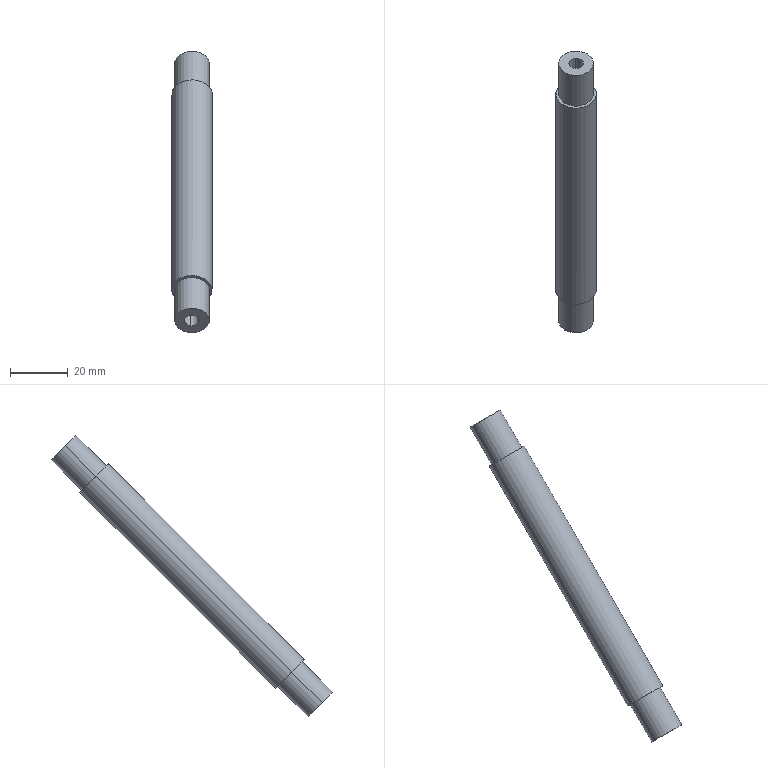Component | SolidWorks | SmallAxisAssembly-1_SmallAxisAssembly1-2_VegetablePressSmallAxis-1 | 1 solid | 18 faces | box 14.05 x 97.58 x 97.58 mm | volume 17562 mm3 | cylinder 10 | cone 4 | plane 4 | commonest cylinder face diameters 5 x4 12 x4 14 x2
build123d program:
from build123d import *

# Parameters (mm, degrees)
M6_TAPPED_HOLE1_D               = 5
M6_TAPPED_HOLE1_DEPTH           = 15
M6_TAPPED_HOLE1_TIP             = 1.502
M6_TAPPED_HOLE1_ON_FACE_2_D     = 5
M6_TAPPED_HOLE1_ON_FACE_2_DEPTH = 15
M6_TAPPED_HOLE1_ON_FACE_2_TIP   = 1.502


with BuildPart() as part:
    # Sketch1 → Revolve1 (revolve)
    with BuildSketch(Plane.XY):
        Polygon((-63, 0), (-63, 6), (-48, 6), (-48, 7), (48, 7), (48, 6), (63, 6), (63, 0), align=None)
    revolve(axis=Axis((63, 0, 0), (-1, 0, 0)))

    # M6 Tapped Hole1
    with Locations(Plane(origin=(63, 0, 0), x_dir=(0, 0, 1), z_dir=(1, 0, 0))):
        with Locations((0, 0)):
            Hole(M6_TAPPED_HOLE1_D / 2, depth=M6_TAPPED_HOLE1_DEPTH)
            with Locations((0, 0, -(M6_TAPPED_HOLE1_DEPTH + M6_TAPPED_HOLE1_TIP / 2))):  # 118° drill point
                Cone(0, M6_TAPPED_HOLE1_D / 2, M6_TAPPED_HOLE1_TIP, mode=Mode.SUBTRACT)

    # M6 Tapped Hole1 on face 2
    with Locations(Plane(origin=(-63, 0, 0), x_dir=(0, 0, -1), z_dir=(-1, 0, 0))):
        with Locations((0, 0)):
            Hole(M6_TAPPED_HOLE1_ON_FACE_2_D / 2, depth=M6_TAPPED_HOLE1_ON_FACE_2_DEPTH)
            with Locations((0, 0, -(M6_TAPPED_HOLE1_ON_FACE_2_DEPTH + M6_TAPPED_HOLE1_ON_FACE_2_TIP / 2))):  # 118° drill point
                Cone(0, M6_TAPPED_HOLE1_ON_FACE_2_D / 2, M6_TAPPED_HOLE1_ON_FACE_2_TIP, mode=Mode.SUBTRACT)


solid = part.part

# Placed as in the assembly
solid = solid.moved(Location((-41.751, 822.318, 226.866), (-135.031, 46.235, -89.957)))
STEP:
#1=COLOUR_RGB('',0.7922,0.8196,0.9333);
#2=FILL_AREA_STYLE_COLOUR('',#1);
#3=FILL_AREA_STYLE('',(#2));
#4=SURFACE_STYLE_FILL_AREA(#3);
#5=SURFACE_SIDE_STYLE('',(#4));
#6=SURFACE_STYLE_USAGE(.BOTH.,#5);
#7=PRESENTATION_STYLE_ASSIGNMENT((#6));
#8=CARTESIAN_POINT('',(-1.657,33.78,10.199));
#9=VERTEX_POINT('',#8);
#10=CARTESIAN_POINT('',(-1.628,33.642,10.337));
#11=VERTEX_POINT('',#10);
#12=CARTESIAN_POINT('',(-1.643,33.711,10.268));
#13=DIRECTION('',(0.0005225,0.7071,0.7071));
#14=DIRECTION('',(0.1474,-0.6994,0.6993));
#15=AXIS2_PLACEMENT_3D('',#12,#13,#14);
#16=CIRCLE('',#15,0.09843);
#17=EDGE_CURVE('',#9,#11,#16,.T.);
#18=ORIENTED_EDGE('',*,*,#17,.F.);
#19=CARTESIAN_POINT('',(-1.657,34.197,10.617));
#20=VERTEX_POINT('',#19);
#21=CARTESIAN_POINT('',(-1.657,34.197,10.617));
#22=DIRECTION('',(0.0005225,0.7071,0.7071));
#23=VECTOR('',#22,39.37);
#24=LINE('',#21,#23);
#25=EDGE_CURVE('',#9,#20,#24,.T.);
#26=ORIENTED_EDGE('',*,*,#25,.T.);
#27=CARTESIAN_POINT('',(-1.628,34.06,10.754));
#28=VERTEX_POINT('',#27);
#29=CARTESIAN_POINT('',(-1.642,34.129,10.686));
#30=DIRECTION('',(0.0005225,0.7071,0.7071));
#31=DIRECTION('',(0.1474,-0.6994,0.6993));
#32=AXIS2_PLACEMENT_3D('',#29,#30,#31);
#33=CIRCLE('',#32,0.09843);
#34=EDGE_CURVE('',#20,#28,#33,.T.);
#35=ORIENTED_EDGE('',*,*,#34,.T.);
#36=CARTESIAN_POINT('',(-1.628,34.06,10.754));
#37=DIRECTION('',(0.0005225,0.7071,0.7071));
#38=VECTOR('',#37,39.37);
#39=LINE('',#36,#38);
#40=EDGE_CURVE('',#11,#28,#39,.T.);
#41=ORIENTED_EDGE('',*,*,#40,.F.);
#42=EDGE_LOOP('',(#18,#26,#35,#41));
#43=FACE_OUTER_BOUND('',#42,.T.);
#44=CARTESIAN_POINT('',(-1.642,34.129,10.686));
#45=DIRECTION('',(0.0005225,0.7071,0.7071));
#46=DIRECTION('',(0.1474,-0.6994,0.6993));
#47=AXIS2_PLACEMENT_3D('',#44,#45,#46);
#48=CYLINDRICAL_SURFACE('',#47,0.09843);
#49=ADVANCED_FACE('',(#43),#48,.F.);
#50=CARTESIAN_POINT('',(-1.643,33.669,10.226));
#51=VERTEX_POINT('',#50);
#52=CARTESIAN_POINT('',(-1.628,33.642,10.337));
#53=DIRECTION('',(0.1266,-0.2353,0.9636));
#54=VECTOR('',#53,39.37);
#55=LINE('',#52,#54);
#56=EDGE_CURVE('',#51,#11,#55,.T.);
#57=ORIENTED_EDGE('',*,*,#56,.F.);
#58=CARTESIAN_POINT('',(-1.657,33.78,10.199));
#59=DIRECTION('',(-0.1261,0.9637,-0.2353));
#60=VECTOR('',#59,39.37);
#61=LINE('',#58,#60);
#62=EDGE_CURVE('',#51,#9,#61,.T.);
#63=ORIENTED_EDGE('',*,*,#62,.T.);
#64=ORIENTED_EDGE('',*,*,#17,.T.);
#65=EDGE_LOOP('',(#57,#63,#64));
#66=FACE_OUTER_BOUND('',#65,.T.);
#67=CARTESIAN_POINT('',(-1.643,33.711,10.268));
#68=DIRECTION('',(0.0005225,0.7071,0.7071));
#69=DIRECTION('',(0.1474,-0.6994,0.6993));
#70=AXIS2_PLACEMENT_3D('',#67,#68,#69);
#71=CONICAL_SURFACE('',#70,0.09843,1.03);
#72=ADVANCED_FACE('',(#66),#71,.F.);
#73=CARTESIAN_POINT('',(-1.63,30.97,7.664));
#74=VERTEX_POINT('',#73);
#75=CARTESIAN_POINT('',(-1.659,31.107,7.527));
#76=VERTEX_POINT('',#75);
#77=CARTESIAN_POINT('',(-1.645,31.038,7.595));
#78=DIRECTION('',(-0.0005225,-0.7071,-0.7071));
#79=DIRECTION('',(-0.1474,0.6994,-0.6993));
#80=AXIS2_PLACEMENT_3D('',#77,#78,#79);
#81=CIRCLE('',#80,0.09843);
#82=EDGE_CURVE('',#74,#76,#81,.T.);
#83=ORIENTED_EDGE('',*,*,#82,.F.);
#84=CARTESIAN_POINT('',(-1.631,30.552,7.247));
#85=VERTEX_POINT('',#84);
#86=CARTESIAN_POINT('',(-1.631,30.552,7.247));
#87=DIRECTION('',(-0.0005225,-0.7071,-0.7071));
#88=VECTOR('',#87,39.37);
#89=LINE('',#86,#88);
#90=EDGE_CURVE('',#74,#85,#89,.T.);
#91=ORIENTED_EDGE('',*,*,#90,.T.);
#92=CARTESIAN_POINT('',(-1.66,30.69,7.109));
#93=VERTEX_POINT('',#92);
#94=CARTESIAN_POINT('',(-1.645,30.621,7.178));
#95=DIRECTION('',(-0.0005225,-0.7071,-0.7071));
#96=DIRECTION('',(-0.1474,0.6994,-0.6993));
#97=AXIS2_PLACEMENT_3D('',#94,#95,#96);
#98=CIRCLE('',#97,0.09843);
#99=EDGE_CURVE('',#85,#93,#98,.T.);
#100=ORIENTED_EDGE('',*,*,#99,.T.);
#101=CARTESIAN_POINT('',(-1.66,30.69,7.109));
#102=DIRECTION('',(-0.0005225,-0.7071,-0.7071));
#103=VECTOR('',#102,39.37);
#104=LINE('',#101,#103);
#105=EDGE_CURVE('',#76,#93,#104,.T.);
#106=ORIENTED_EDGE('',*,*,#105,.F.);
#107=EDGE_LOOP('',(#83,#91,#100,#106));
#108=FACE_OUTER_BOUND('',#107,.T.);
#109=CARTESIAN_POINT('',(-1.645,30.621,7.178));
#110=DIRECTION('',(-0.0005225,-0.7071,-0.7071));
#111=DIRECTION('',(-0.1474,0.6994,-0.6993));
#112=AXIS2_PLACEMENT_3D('',#109,#110,#111);
#113=CYLINDRICAL_SURFACE('',#112,0.09843);
#114=ADVANCED_FACE('',(#108),#113,.F.);
#115=CARTESIAN_POINT('',(-1.645,31.08,7.637));
#116=VERTEX_POINT('',#115);
#117=CARTESIAN_POINT('',(-1.659,31.107,7.527));
#118=DIRECTION('',(-0.1266,0.2353,-0.9636));
#119=VECTOR('',#118,39.37);
#120=LINE('',#117,#119);
#121=EDGE_CURVE('',#116,#76,#120,.T.);
#122=ORIENTED_EDGE('',*,*,#121,.F.);
#123=CARTESIAN_POINT('',(-1.63,30.97,7.664));
#124=DIRECTION('',(0.1261,-0.9637,0.2353));
#125=VECTOR('',#124,39.37);
#126=LINE('',#123,#125);
#127=EDGE_CURVE('',#116,#74,#126,.T.);
#128=ORIENTED_EDGE('',*,*,#127,.T.);
#129=ORIENTED_EDGE('',*,*,#82,.T.);
#130=EDGE_LOOP('',(#122,#128,#129));
#131=FACE_OUTER_BOUND('',#130,.T.);
#132=CARTESIAN_POINT('',(-1.645,31.038,7.595));
#133=DIRECTION('',(-0.0005225,-0.7071,-0.7071));
#134=DIRECTION('',(-0.1474,0.6994,-0.6993));
#135=AXIS2_PLACEMENT_3D('',#132,#133,#134);
#136=CONICAL_SURFACE('',#135,0.09843,1.03);
#137=ADVANCED_FACE('',(#131),#136,.F.);
#138=CARTESIAN_POINT('',(-1.409,33.736,10.243));
#139=VERTEX_POINT('',#138);
#140=CARTESIAN_POINT('',(-1.876,33.686,10.293));
#141=VERTEX_POINT('',#140);
#142=CARTESIAN_POINT('',(-1.643,33.711,10.268));
#143=DIRECTION('',(0.0005225,0.7071,0.7071));
#144=DIRECTION('',(0.9891,0.1039,-0.1046));
#145=AXIS2_PLACEMENT_3D('',#142,#143,#144);
#146=CIRCLE('',#145,0.2362);
#147=EDGE_CURVE('',#139,#141,#146,.T.);
#148=ORIENTED_EDGE('',*,*,#147,.T.);
#149=CARTESIAN_POINT('',(-1.876,34.104,10.71));
#150=VERTEX_POINT('',#149);
#151=CARTESIAN_POINT('',(-1.876,34.104,10.71));
#152=DIRECTION('',(0.0005225,0.7071,0.7071));
#153=VECTOR('',#152,39.37);
#154=LINE('',#151,#153);
#155=EDGE_CURVE('',#141,#150,#154,.T.);
#156=ORIENTED_EDGE('',*,*,#155,.T.);
#157=CARTESIAN_POINT('',(-1.409,34.153,10.661));
#158=VERTEX_POINT('',#157);
#159=CARTESIAN_POINT('',(-1.642,34.129,10.686));
#160=DIRECTION('',(0.0005225,0.7071,0.7071));
#161=DIRECTION('',(0.9891,0.1039,-0.1046));
#162=AXIS2_PLACEMENT_3D('',#159,#160,#161);
#163=CIRCLE('',#162,0.2362);
#164=EDGE_CURVE('',#158,#150,#163,.T.);
#165=ORIENTED_EDGE('',*,*,#164,.F.);
#166=CARTESIAN_POINT('',(-1.409,34.153,10.661));
#167=DIRECTION('',(0.0005225,0.7071,0.7071));
#168=VECTOR('',#167,39.37);
#169=LINE('',#166,#168);
#170=EDGE_CURVE('',#139,#158,#169,.T.);
#171=ORIENTED_EDGE('',*,*,#170,.F.);
#172=EDGE_LOOP('',(#148,#156,#165,#171));
#173=FACE_OUTER_BOUND('',#172,.T.);
#174=CARTESIAN_POINT('',(-1.642,34.129,10.686));
#175=DIRECTION('',(0.0005225,0.7071,0.7071));
#176=DIRECTION('',(0.9891,0.1039,-0.1046));
#177=AXIS2_PLACEMENT_3D('',#174,#175,#176);
#178=CYLINDRICAL_SURFACE('',#177,0.2362);
#179=ADVANCED_FACE('',(#173),#178,.T.);
#180=CARTESIAN_POINT('',(-1.372,31.067,7.567));
#181=VERTEX_POINT('',#180);
#182=CARTESIAN_POINT('',(-1.917,31.01,7.624));
#183=VERTEX_POINT('',#182);
#184=CARTESIAN_POINT('',(-1.645,31.038,7.595));
#185=DIRECTION('',(0.0005225,0.7071,0.7071));
#186=DIRECTION('',(0.9891,0.1039,-0.1046));
#187=AXIS2_PLACEMENT_3D('',#184,#185,#186);
#188=CIRCLE('',#187,0.2756);
#189=EDGE_CURVE('',#181,#183,#188,.T.);
#190=ORIENTED_EDGE('',*,*,#189,.T.);
#191=CARTESIAN_POINT('',(-1.915,33.682,10.297));
#192=VERTEX_POINT('',#191);
#193=CARTESIAN_POINT('',(-1.915,34.1,10.714));
#194=DIRECTION('',(0.0005225,0.7071,0.7071));
#195=VECTOR('',#194,39.37);
#196=LINE('',#193,#195);
#197=EDGE_CURVE('',#183,#192,#196,.T.);
#198=ORIENTED_EDGE('',*,*,#197,.T.);
#199=CARTESIAN_POINT('',(-1.37,33.74,10.239));
#200=VERTEX_POINT('',#199);
#201=CARTESIAN_POINT('',(-1.643,33.711,10.268));
#202=DIRECTION('',(0.0005225,0.7071,0.7071));
#203=DIRECTION('',(0.9891,0.1039,-0.1046));
#204=AXIS2_PLACEMENT_3D('',#201,#202,#203);
#205=CIRCLE('',#204,0.2756);
#206=EDGE_CURVE('',#200,#192,#205,.T.);
#207=ORIENTED_EDGE('',*,*,#206,.F.);
#208=CARTESIAN_POINT('',(-1.37,34.157,10.657));
#209=DIRECTION('',(0.0005225,0.7071,0.7071));
#210=VECTOR('',#209,39.37);
#211=LINE('',#208,#210);
#212=EDGE_CURVE('',#181,#200,#211,.T.);
#213=ORIENTED_EDGE('',*,*,#212,.F.);
#214=EDGE_LOOP('',(#190,#198,#207,#213));
#215=FACE_OUTER_BOUND('',#214,.T.);
#216=CARTESIAN_POINT('',(-1.642,34.129,10.686));
#217=DIRECTION('',(0.0005225,0.7071,0.7071));
#218=DIRECTION('',(0.9891,0.1039,-0.1046));
#219=AXIS2_PLACEMENT_3D('',#216,#217,#218);
#220=CYLINDRICAL_SURFACE('',#219,0.2756);
#221=ADVANCED_FACE('',(#215),#220,.T.);
#222=CARTESIAN_POINT('',(-1.411,30.645,7.153));
#223=VERTEX_POINT('',#222);
#224=CARTESIAN_POINT('',(-1.879,30.596,7.203));
#225=VERTEX_POINT('',#224);
#226=CARTESIAN_POINT('',(-1.645,30.621,7.178));
#227=DIRECTION('',(0.0005225,0.7071,0.7071));
#228=DIRECTION('',(0.9891,0.1039,-0.1046));
#229=AXIS2_PLACEMENT_3D('',#226,#227,#228);
#230=CIRCLE('',#229,0.2362);
#231=EDGE_CURVE('',#223,#225,#230,.T.);
#232=ORIENTED_EDGE('',*,*,#231,.T.);
#233=CARTESIAN_POINT('',(-1.878,31.014,7.62));
#234=VERTEX_POINT('',#233);
#235=CARTESIAN_POINT('',(-1.876,34.104,10.71));
#236=DIRECTION('',(0.0005225,0.7071,0.7071));
#237=VECTOR('',#236,39.37);
#238=LINE('',#235,#237);
#239=EDGE_CURVE('',#225,#234,#238,.T.);
#240=ORIENTED_EDGE('',*,*,#239,.T.);
#241=CARTESIAN_POINT('',(-1.411,31.063,7.571));
#242=VERTEX_POINT('',#241);
#243=CARTESIAN_POINT('',(-1.645,31.038,7.595));
#244=DIRECTION('',(0.0005225,0.7071,0.7071));
#245=DIRECTION('',(0.9891,0.1039,-0.1046));
#246=AXIS2_PLACEMENT_3D('',#243,#244,#245);
#247=CIRCLE('',#246,0.2362);
#248=EDGE_CURVE('',#242,#234,#247,.T.);
#249=ORIENTED_EDGE('',*,*,#248,.F.);
#250=CARTESIAN_POINT('',(-1.409,34.153,10.661));
#251=DIRECTION('',(0.0005225,0.7071,0.7071));
#252=VECTOR('',#251,39.37);
#253=LINE('',#250,#252);
#254=EDGE_CURVE('',#223,#242,#253,.T.);
#255=ORIENTED_EDGE('',*,*,#254,.F.);
#256=EDGE_LOOP('',(#232,#240,#249,#255));
#257=FACE_OUTER_BOUND('',#256,.T.);
#258=CARTESIAN_POINT('',(-1.642,34.129,10.686));
#259=DIRECTION('',(0.0005225,0.7071,0.7071));
#260=DIRECTION('',(0.9891,0.1039,-0.1046));
#261=AXIS2_PLACEMENT_3D('',#258,#259,#260);
#262=CYLINDRICAL_SURFACE('',#261,0.2362);
#263=ADVANCED_FACE('',(#257),#262,.T.);
#264=CARTESIAN_POINT('',(-1.645,30.621,7.178));
#265=DIRECTION('',(-0.0005225,-0.7071,-0.7071));
#266=DIRECTION('',(-0.1474,0.6994,-0.6993));
#267=AXIS2_PLACEMENT_3D('',#264,#265,#266);
#268=CIRCLE('',#267,0.09843);
#269=EDGE_CURVE('',#93,#85,#268,.T.);
#270=ORIENTED_EDGE('',*,*,#269,.F.);
#271=ORIENTED_EDGE('',*,*,#99,.F.);
#272=EDGE_LOOP('',(#270,#271));
#273=FACE_BOUND('',#272,.T.);
#274=ORIENTED_EDGE('',*,*,#231,.F.);
#275=CARTESIAN_POINT('',(-1.645,30.621,7.178));
#276=DIRECTION('',(0.0005225,0.7071,0.7071));
#277=DIRECTION('',(0.9891,0.1039,-0.1046));
#278=AXIS2_PLACEMENT_3D('',#275,#276,#277);
#279=CIRCLE('',#278,0.2362);
#280=EDGE_CURVE('',#225,#223,#279,.T.);
#281=ORIENTED_EDGE('',*,*,#280,.F.);
#282=EDGE_LOOP('',(#274,#281));
#283=FACE_OUTER_BOUND('',#282,.T.);
#284=CARTESIAN_POINT('',(-1.645,30.621,7.178));
#285=DIRECTION('',(-0.0005225,-0.7071,-0.7071));
#286=DIRECTION('',(-0.9891,-0.1039,0.1046));
#287=AXIS2_PLACEMENT_3D('',#284,#285,#286);
#288=PLANE('',#287);
#289=ADVANCED_FACE('',(#273,#283),#288,.T.);
#290=ORIENTED_EDGE('',*,*,#239,.F.);
#291=ORIENTED_EDGE('',*,*,#280,.T.);
#292=ORIENTED_EDGE('',*,*,#254,.T.);
#293=CARTESIAN_POINT('',(-1.645,31.038,7.595));
#294=DIRECTION('',(0.0005225,0.7071,0.7071));
#295=DIRECTION('',(0.9891,0.1039,-0.1046));
#296=AXIS2_PLACEMENT_3D('',#293,#294,#295);
#297=CIRCLE('',#296,0.2362);
#298=EDGE_CURVE('',#234,#242,#297,.T.);
#299=ORIENTED_EDGE('',*,*,#298,.F.);
#300=EDGE_LOOP('',(#290,#291,#292,#299));
#301=FACE_OUTER_BOUND('',#300,.T.);
#302=CARTESIAN_POINT('',(-1.642,34.129,10.686));
#303=DIRECTION('',(0.0005225,0.7071,0.7071));
#304=DIRECTION('',(0.9891,0.1039,-0.1046));
#305=AXIS2_PLACEMENT_3D('',#302,#303,#304);
#306=CYLINDRICAL_SURFACE('',#305,0.2362);
#307=ADVANCED_FACE('',(#301),#306,.T.);
#308=ORIENTED_EDGE('',*,*,#248,.T.);
#309=ORIENTED_EDGE('',*,*,#298,.T.);
#310=EDGE_LOOP('',(#308,#309));
#311=FACE_BOUND('',#310,.T.);
#312=ORIENTED_EDGE('',*,*,#189,.F.);
#313=CARTESIAN_POINT('',(-1.645,31.038,7.595));
#314=DIRECTION('',(0.0005225,0.7071,0.7071));
#315=DIRECTION('',(0.9891,0.1039,-0.1046));
#316=AXIS2_PLACEMENT_3D('',#313,#314,#315);
#317=CIRCLE('',#316,0.2756);
#318=EDGE_CURVE('',#183,#181,#317,.T.);
#319=ORIENTED_EDGE('',*,*,#318,.F.);
#320=EDGE_LOOP('',(#312,#319));
#321=FACE_OUTER_BOUND('',#320,.T.);
#322=CARTESIAN_POINT('',(-1.411,31.063,7.571));
#323=DIRECTION('',(-0.0005225,-0.7071,-0.7071));
#324=DIRECTION('',(-0.9891,-0.1039,0.1046));
#325=AXIS2_PLACEMENT_3D('',#322,#323,#324);
#326=PLANE('',#325);
#327=ADVANCED_FACE('',(#311,#321),#326,.T.);
#328=ORIENTED_EDGE('',*,*,#197,.F.);
#329=ORIENTED_EDGE('',*,*,#318,.T.);
#330=ORIENTED_EDGE('',*,*,#212,.T.);
#331=CARTESIAN_POINT('',(-1.643,33.711,10.268));
#332=DIRECTION('',(0.0005225,0.7071,0.7071));
#333=DIRECTION('',(0.9891,0.1039,-0.1046));
#334=AXIS2_PLACEMENT_3D('',#331,#332,#333);
#335=CIRCLE('',#334,0.2756);
#336=EDGE_CURVE('',#192,#200,#335,.T.);
#337=ORIENTED_EDGE('',*,*,#336,.F.);
#338=EDGE_LOOP('',(#328,#329,#330,#337));
#339=FACE_OUTER_BOUND('',#338,.T.);
#340=CARTESIAN_POINT('',(-1.642,34.129,10.686));
#341=DIRECTION('',(0.0005225,0.7071,0.7071));
#342=DIRECTION('',(0.9891,0.1039,-0.1046));
#343=AXIS2_PLACEMENT_3D('',#340,#341,#342);
#344=CYLINDRICAL_SURFACE('',#343,0.2756);
#345=ADVANCED_FACE('',(#339),#344,.T.);
#346=ORIENTED_EDGE('',*,*,#206,.T.);
#347=ORIENTED_EDGE('',*,*,#336,.T.);
#348=EDGE_LOOP('',(#346,#347));
#349=FACE_OUTER_BOUND('',#348,.T.);
#350=ORIENTED_EDGE('',*,*,#147,.F.);
#351=CARTESIAN_POINT('',(-1.643,33.711,10.268));
#352=DIRECTION('',(0.0005225,0.7071,0.7071));
#353=DIRECTION('',(0.9891,0.1039,-0.1046));
#354=AXIS2_PLACEMENT_3D('',#351,#352,#353);
#355=CIRCLE('',#354,0.2362);
#356=EDGE_CURVE('',#141,#139,#355,.T.);
#357=ORIENTED_EDGE('',*,*,#356,.F.);
#358=EDGE_LOOP('',(#350,#357));
#359=FACE_BOUND('',#358,.T.);
#360=CARTESIAN_POINT('',(-1.37,33.74,10.239));
#361=DIRECTION('',(0.0005225,0.7071,0.7071));
#362=DIRECTION('',(0.9891,0.1039,-0.1046));
#363=AXIS2_PLACEMENT_3D('',#360,#361,#362);
#364=PLANE('',#363);
#365=ADVANCED_FACE('',(#349,#359),#364,.T.);
#366=ORIENTED_EDGE('',*,*,#155,.F.);
#367=ORIENTED_EDGE('',*,*,#356,.T.);
#368=ORIENTED_EDGE('',*,*,#170,.T.);
#369=CARTESIAN_POINT('',(-1.642,34.129,10.686));
#370=DIRECTION('',(0.0005225,0.7071,0.7071));
#371=DIRECTION('',(0.9891,0.1039,-0.1046));
#372=AXIS2_PLACEMENT_3D('',#369,#370,#371);
#373=CIRCLE('',#372,0.2362);
#374=EDGE_CURVE('',#150,#158,#373,.T.);
#375=ORIENTED_EDGE('',*,*,#374,.F.);
#376=EDGE_LOOP('',(#366,#367,#368,#375));
#377=FACE_OUTER_BOUND('',#376,.T.);
#378=CARTESIAN_POINT('',(-1.642,34.129,10.686));
#379=DIRECTION('',(0.0005225,0.7071,0.7071));
#380=DIRECTION('',(0.9891,0.1039,-0.1046));
#381=AXIS2_PLACEMENT_3D('',#378,#379,#380);
#382=CYLINDRICAL_SURFACE('',#381,0.2362);
#383=ADVANCED_FACE('',(#377),#382,.T.);
#384=CARTESIAN_POINT('',(-1.642,34.129,10.686));
#385=DIRECTION('',(0.0005225,0.7071,0.7071));
#386=DIRECTION('',(0.1474,-0.6994,0.6993));
#387=AXIS2_PLACEMENT_3D('',#384,#385,#386);
#388=CIRCLE('',#387,0.09843);
#389=EDGE_CURVE('',#28,#20,#388,.T.);
#390=ORIENTED_EDGE('',*,*,#389,.F.);
#391=ORIENTED_EDGE('',*,*,#34,.F.);
#392=EDGE_LOOP('',(#390,#391));
#393=FACE_BOUND('',#392,.T.);
#394=ORIENTED_EDGE('',*,*,#164,.T.);
#395=ORIENTED_EDGE('',*,*,#374,.T.);
#396=EDGE_LOOP('',(#394,#395));
#397=FACE_OUTER_BOUND('',#396,.T.);
#398=CARTESIAN_POINT('',(-1.409,34.153,10.661));
#399=DIRECTION('',(0.0005225,0.7071,0.7071));
#400=DIRECTION('',(0.9891,0.1039,-0.1046));
#401=AXIS2_PLACEMENT_3D('',#398,#399,#400);
#402=PLANE('',#401);
#403=ADVANCED_FACE('',(#393,#397),#402,.T.);
#404=ORIENTED_EDGE('',*,*,#127,.F.);
#405=ORIENTED_EDGE('',*,*,#121,.T.);
#406=CARTESIAN_POINT('',(-1.645,31.038,7.595));
#407=DIRECTION('',(-0.0005225,-0.7071,-0.7071));
#408=DIRECTION('',(-0.1474,0.6994,-0.6993));
#409=AXIS2_PLACEMENT_3D('',#406,#407,#408);
#410=CIRCLE('',#409,0.09843);
#411=EDGE_CURVE('',#76,#74,#410,.T.);
#412=ORIENTED_EDGE('',*,*,#411,.T.);
#413=EDGE_LOOP('',(#404,#405,#412));
#414=FACE_OUTER_BOUND('',#413,.T.);
#415=CARTESIAN_POINT('',(-1.645,31.038,7.595));
#416=DIRECTION('',(-0.0005225,-0.7071,-0.7071));
#417=DIRECTION('',(-0.1474,0.6994,-0.6993));
#418=AXIS2_PLACEMENT_3D('',#415,#416,#417);
#419=CONICAL_SURFACE('',#418,0.09843,1.03);
#420=ADVANCED_FACE('',(#414),#419,.F.);
#421=ORIENTED_EDGE('',*,*,#90,.F.);
#422=ORIENTED_EDGE('',*,*,#411,.F.);
#423=ORIENTED_EDGE('',*,*,#105,.T.);
#424=ORIENTED_EDGE('',*,*,#269,.T.);
#425=EDGE_LOOP('',(#421,#422,#423,#424));
#426=FACE_OUTER_BOUND('',#425,.T.);
#427=CARTESIAN_POINT('',(-1.645,30.621,7.178));
#428=DIRECTION('',(-0.0005225,-0.7071,-0.7071));
#429=DIRECTION('',(-0.1474,0.6994,-0.6993));
#430=AXIS2_PLACEMENT_3D('',#427,#428,#429);
#431=CYLINDRICAL_SURFACE('',#430,0.09843);
#432=ADVANCED_FACE('',(#426),#431,.F.);
#433=ORIENTED_EDGE('',*,*,#62,.F.);
#434=ORIENTED_EDGE('',*,*,#56,.T.);
#435=CARTESIAN_POINT('',(-1.643,33.711,10.268));
#436=DIRECTION('',(0.0005225,0.7071,0.7071));
#437=DIRECTION('',(0.1474,-0.6994,0.6993));
#438=AXIS2_PLACEMENT_3D('',#435,#436,#437);
#439=CIRCLE('',#438,0.09843);
#440=EDGE_CURVE('',#11,#9,#439,.T.);
#441=ORIENTED_EDGE('',*,*,#440,.T.);
#442=EDGE_LOOP('',(#433,#434,#441));
#443=FACE_OUTER_BOUND('',#442,.T.);
#444=CARTESIAN_POINT('',(-1.643,33.711,10.268));
#445=DIRECTION('',(0.0005225,0.7071,0.7071));
#446=DIRECTION('',(0.1474,-0.6994,0.6993));
#447=AXIS2_PLACEMENT_3D('',#444,#445,#446);
#448=CONICAL_SURFACE('',#447,0.09843,1.03);
#449=ADVANCED_FACE('',(#443),#448,.F.);
#450=ORIENTED_EDGE('',*,*,#25,.F.);
#451=ORIENTED_EDGE('',*,*,#440,.F.);
#452=ORIENTED_EDGE('',*,*,#40,.T.);
#453=ORIENTED_EDGE('',*,*,#389,.T.);
#454=EDGE_LOOP('',(#450,#451,#452,#453));
#455=FACE_OUTER_BOUND('',#454,.T.);
#456=CARTESIAN_POINT('',(-1.642,34.129,10.686));
#457=DIRECTION('',(0.0005225,0.7071,0.7071));
#458=DIRECTION('',(0.1474,-0.6994,0.6993));
#459=AXIS2_PLACEMENT_3D('',#456,#457,#458);
#460=CYLINDRICAL_SURFACE('',#459,0.09843);
#461=ADVANCED_FACE('',(#455),#460,.F.);
#462=CLOSED_SHELL('',(#49,#72,#114,#137,#179,#221,#263,#289,#307,#327,#345,#365,#383,#403,#420,#432,#449,#461));
#463=MANIFOLD_SOLID_BREP('',#462);
#464=STYLED_ITEM('',(#7),#463);
#465=PRESENTATION_LAYER_ASSIGNMENT('','',(#464));
#466=(LENGTH_UNIT()NAMED_UNIT(*)SI_UNIT($,.METRE.));
#467=LENGTH_MEASURE_WITH_UNIT(LENGTH_MEASURE(0.0254),#466);
#468=DIMENSIONAL_EXPONENTS(1.,0.,0.,0.,0.,0.,0.);
#469=(CONVERSION_BASED_UNIT('',#467)LENGTH_UNIT()NAMED_UNIT(#468));
#470=UNCERTAINTY_MEASURE_WITH_UNIT(LENGTH_MEASURE(0.00001),#469,'','');
#471=(NAMED_UNIT(*)PLANE_ANGLE_UNIT()SI_UNIT($,.RADIAN.));
#472=(NAMED_UNIT(*)SI_UNIT($,.STERADIAN.)SOLID_ANGLE_UNIT());
#473=(GEOMETRIC_REPRESENTATION_CONTEXT(3)GLOBAL_UNCERTAINTY_ASSIGNED_CONTEXT((#470))GLOBAL_UNIT_ASSIGNED_CONTEXT((#469,#471,#472))REPRESENTATION_CONTEXT('',''));
#474=MECHANICAL_DESIGN_GEOMETRIC_PRESENTATION_REPRESENTATION('',(#464),#473);
#475=CARTESIAN_POINT('',(0.,0.,0.));
#476=DIRECTION('',(0.,0.,1.));
#477=DIRECTION('',(1.,0.,0.));
#478=AXIS2_PLACEMENT_3D('',#475,#476,#477);
#479=(LENGTH_UNIT()NAMED_UNIT(*)SI_UNIT($,.METRE.));
#480=LENGTH_MEASURE_WITH_UNIT(LENGTH_MEASURE(0.0254),#479);
#481=DIMENSIONAL_EXPONENTS(1.,0.,0.,0.,0.,0.,0.);
#482=(CONVERSION_BASED_UNIT('',#480)LENGTH_UNIT()NAMED_UNIT(#481));
#483=UNCERTAINTY_MEASURE_WITH_UNIT(LENGTH_MEASURE(0.00001),#482,'','');
#484=(NAMED_UNIT(*)PLANE_ANGLE_UNIT()SI_UNIT($,.RADIAN.));
#485=(NAMED_UNIT(*)SI_UNIT($,.STERADIAN.)SOLID_ANGLE_UNIT());
#486=(GEOMETRIC_REPRESENTATION_CONTEXT(3)GLOBAL_UNCERTAINTY_ASSIGNED_CONTEXT((#483))GLOBAL_UNIT_ASSIGNED_CONTEXT((#482,#484,#485))REPRESENTATION_CONTEXT('',''));
#487=ADVANCED_BREP_SHAPE_REPRESENTATION('',(#463,#478),#486);